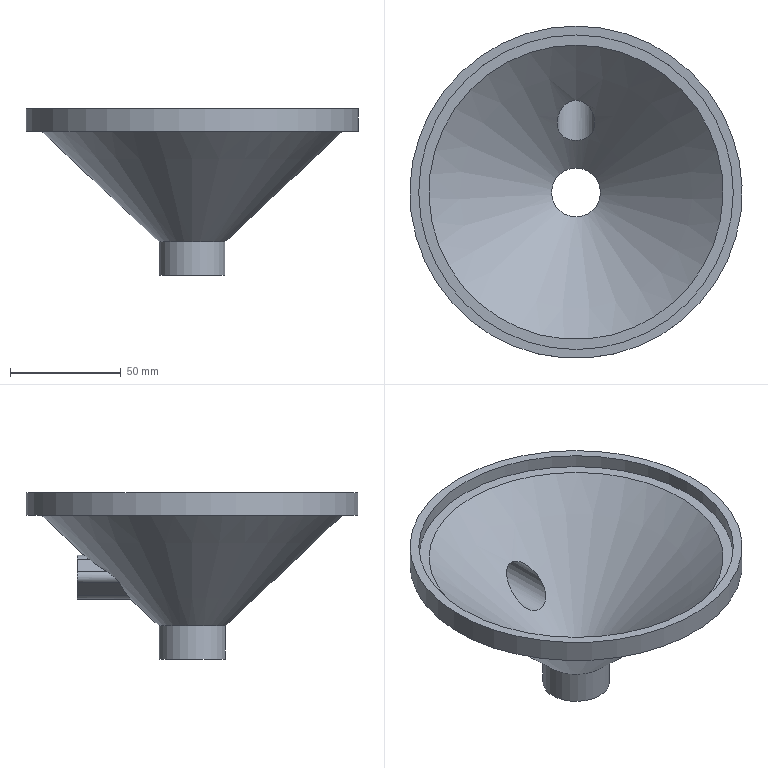Component | NX | 1 | 1 solid | 28 faces | volume 106328 mm3 | cylinder 13 | plane 11 | cone 4 | commonest cylinder face diameters 6 x2 20 x2 2 x2 1.6 x2 150 x1 30 x1 142 x1 22 x1